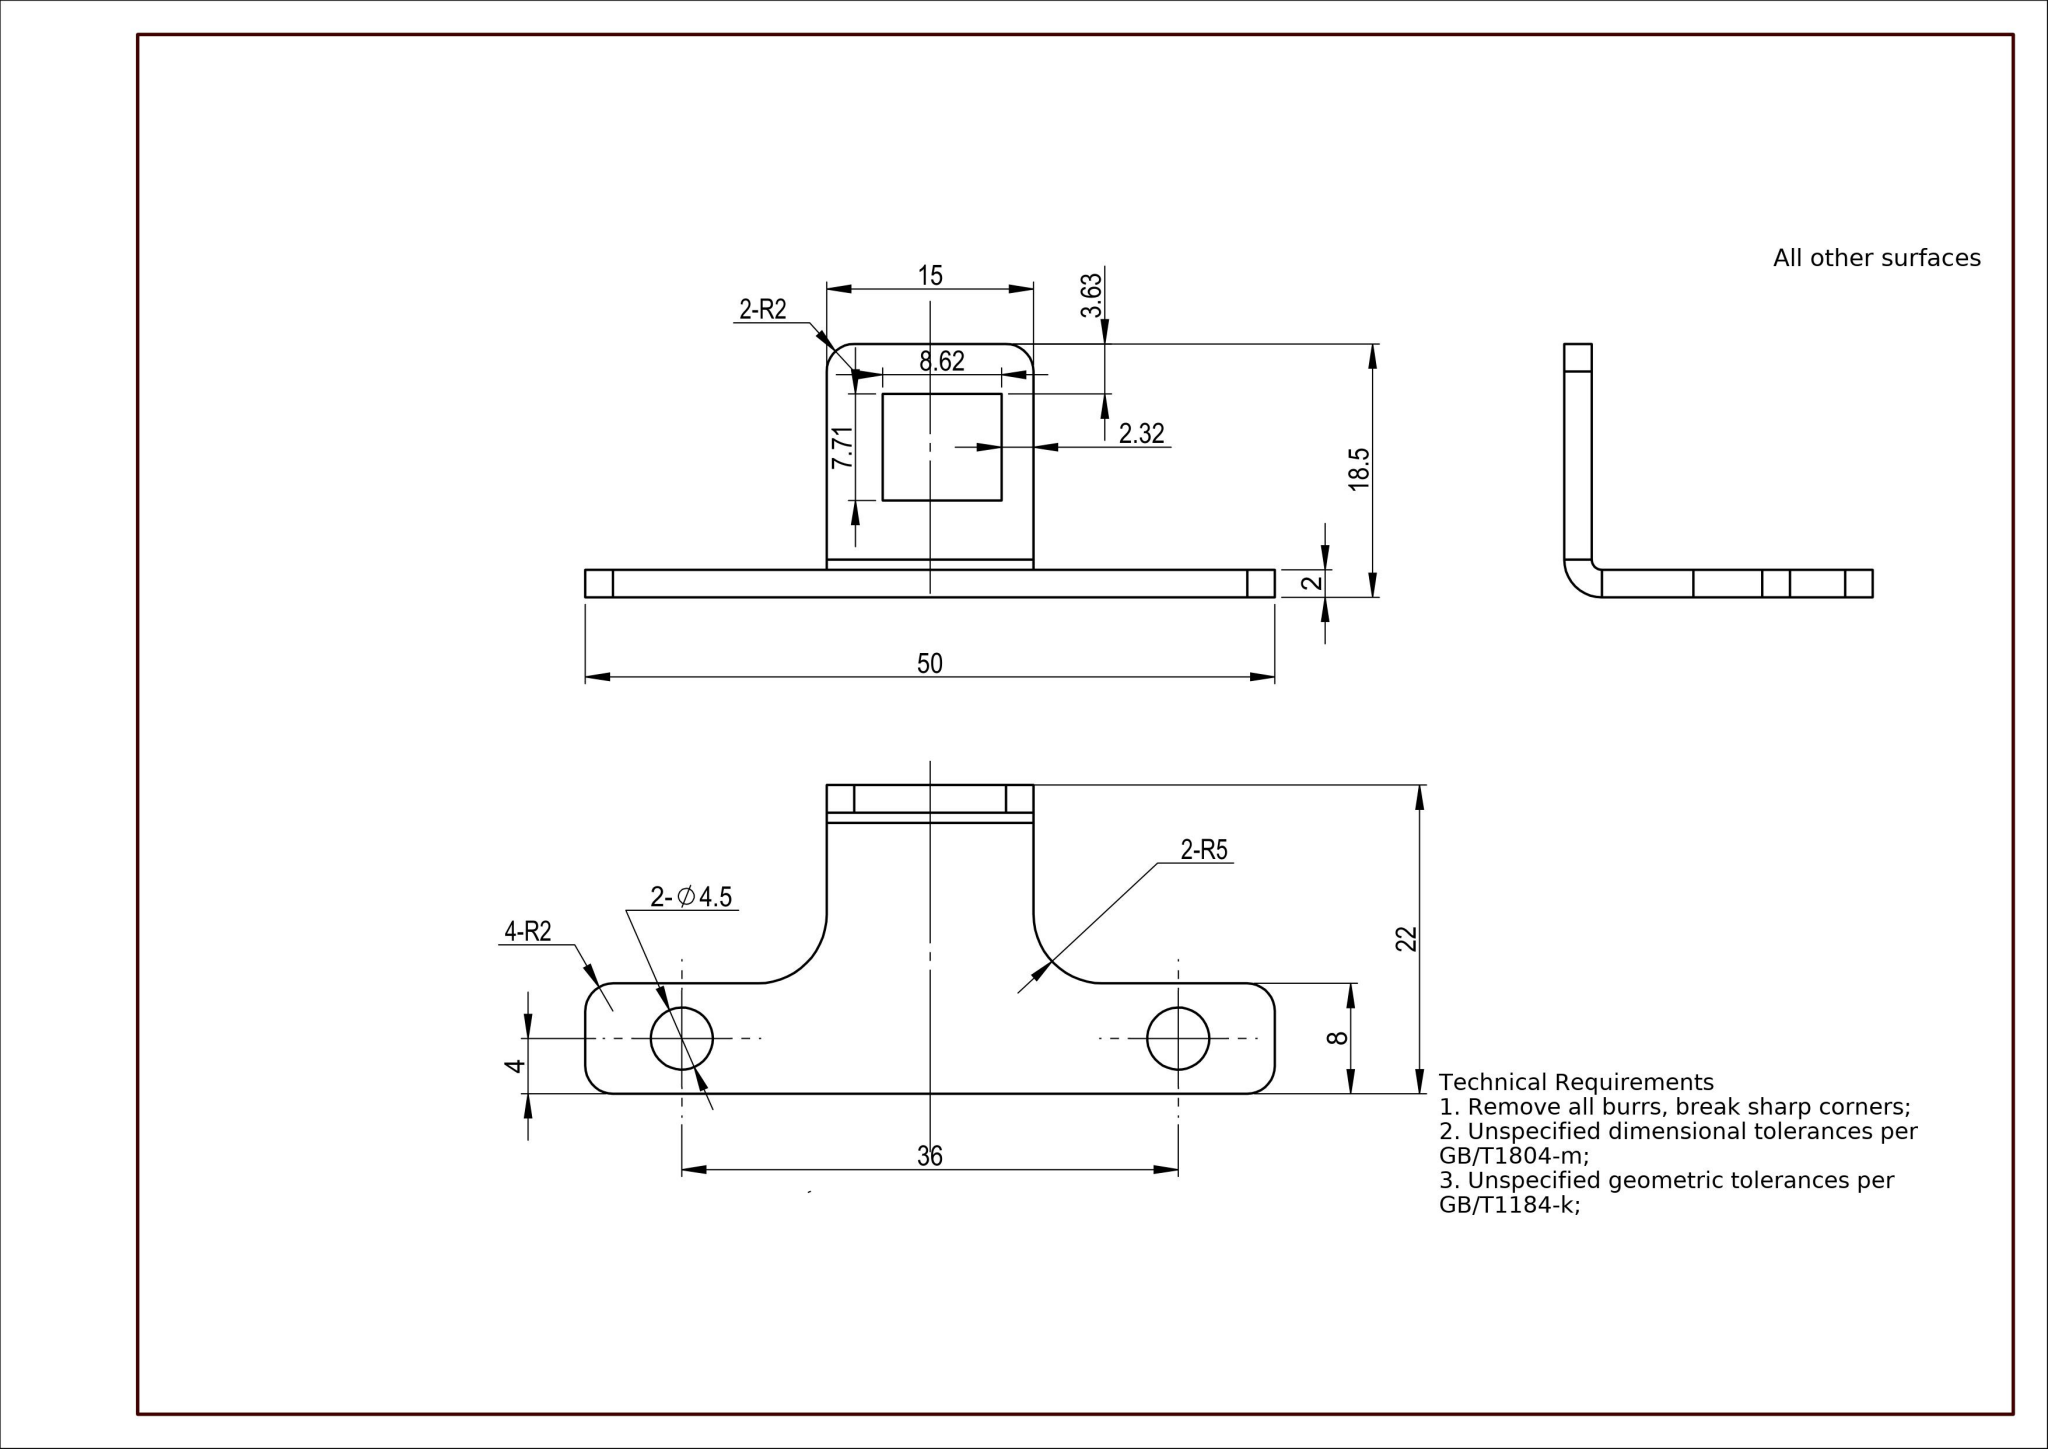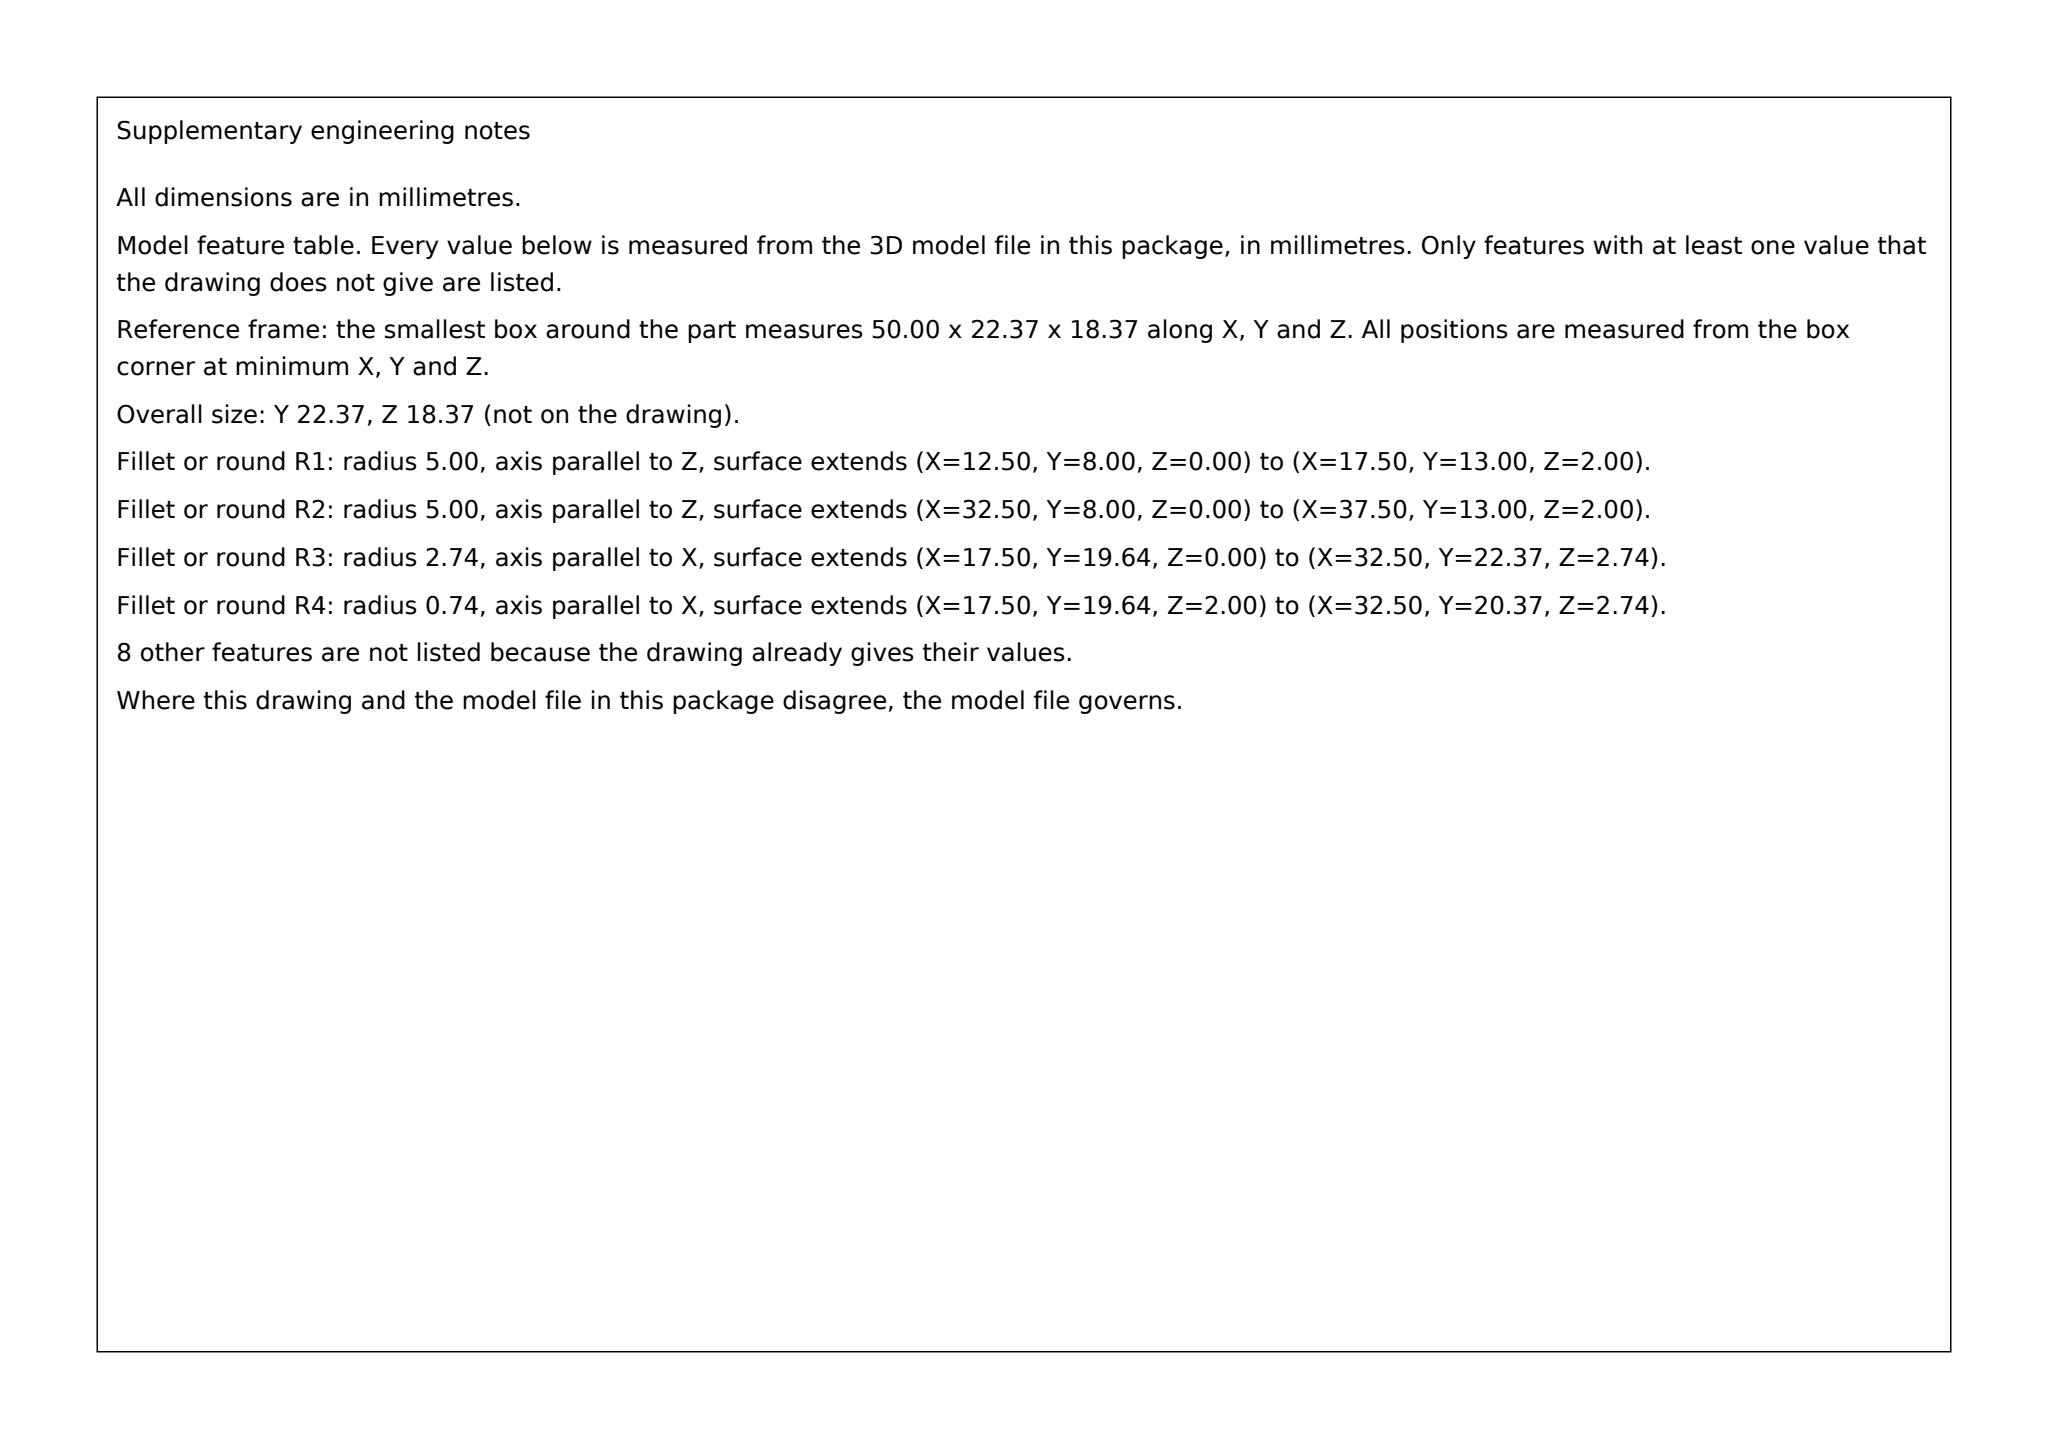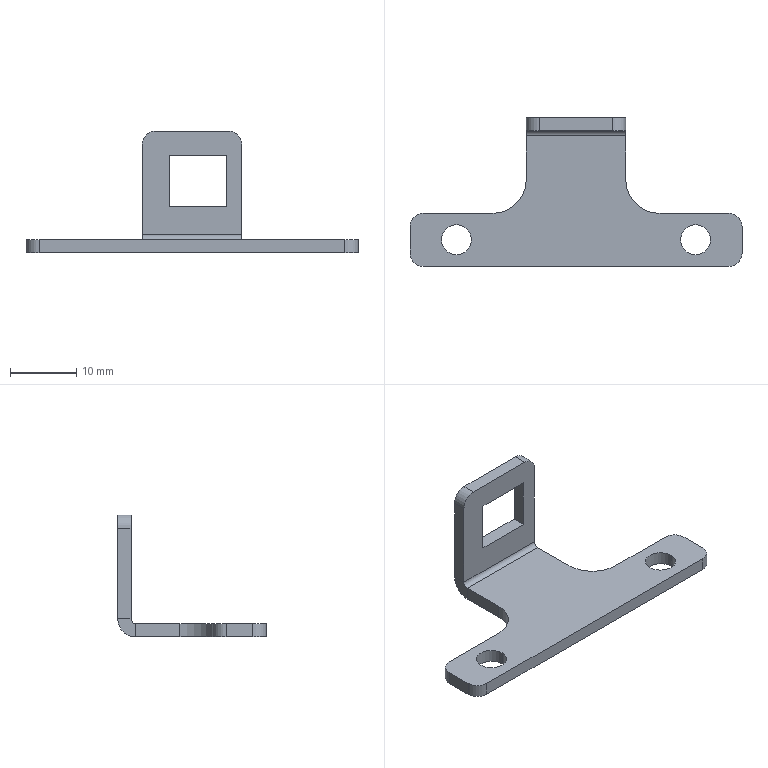Part | SolidWorks | mm | 1 solid | 34 faces | box 50 x 22.37 x 18.37 mm | volume 1514 mm3 | plane 20 | cylinder 14 | commonest cylinder face diameters 4 x6 4.5 x4 10 x2 5.473 x1 1.473 x1